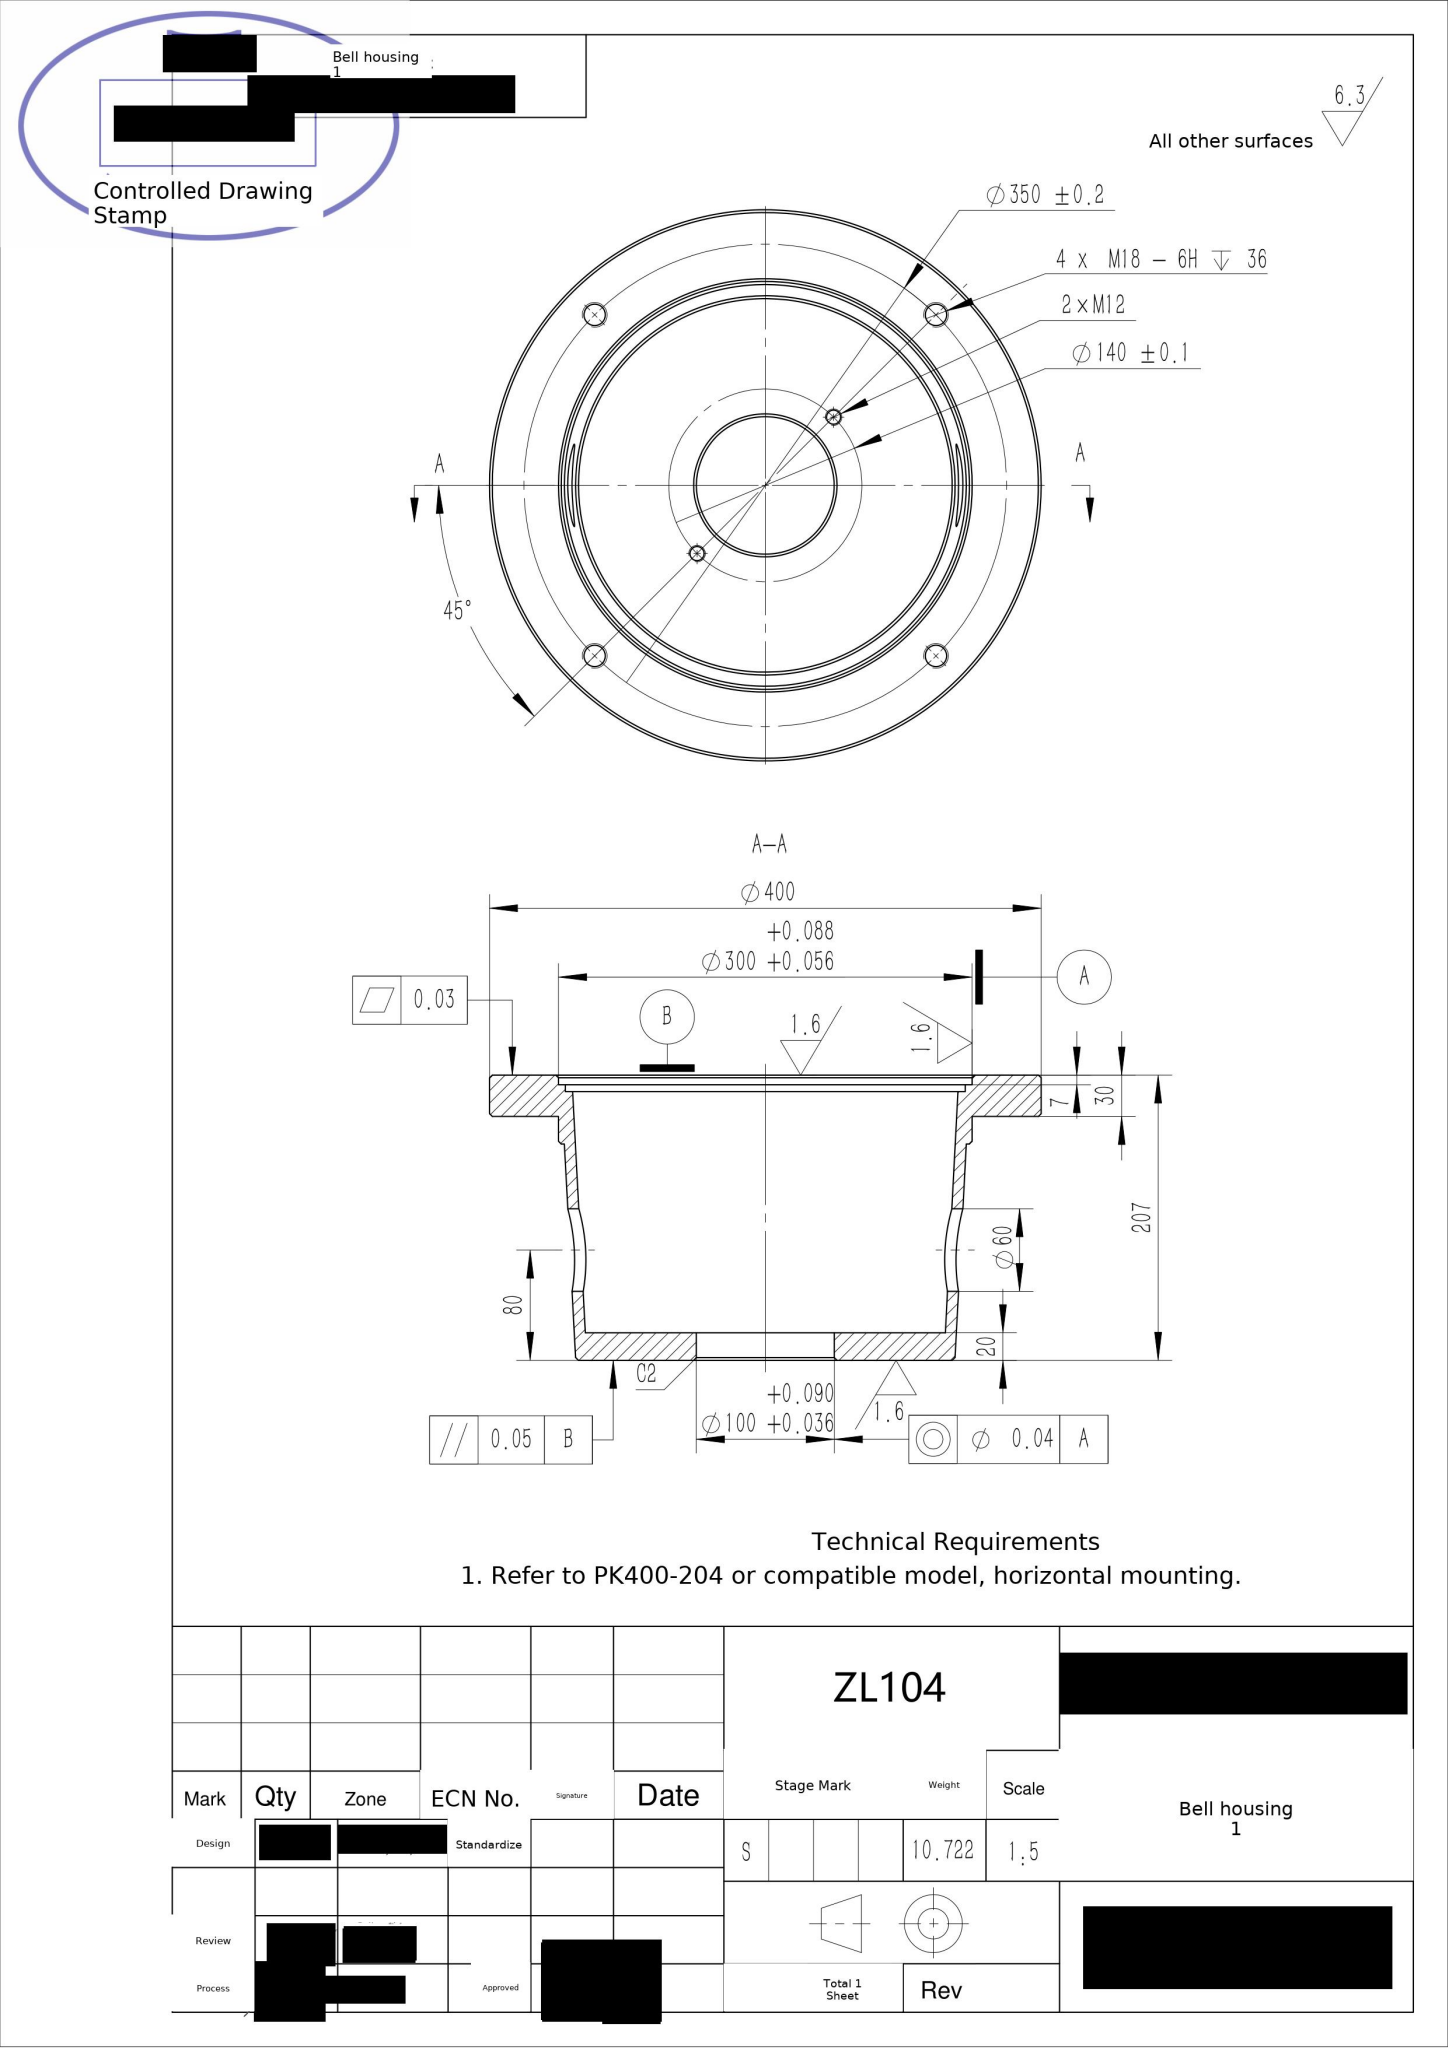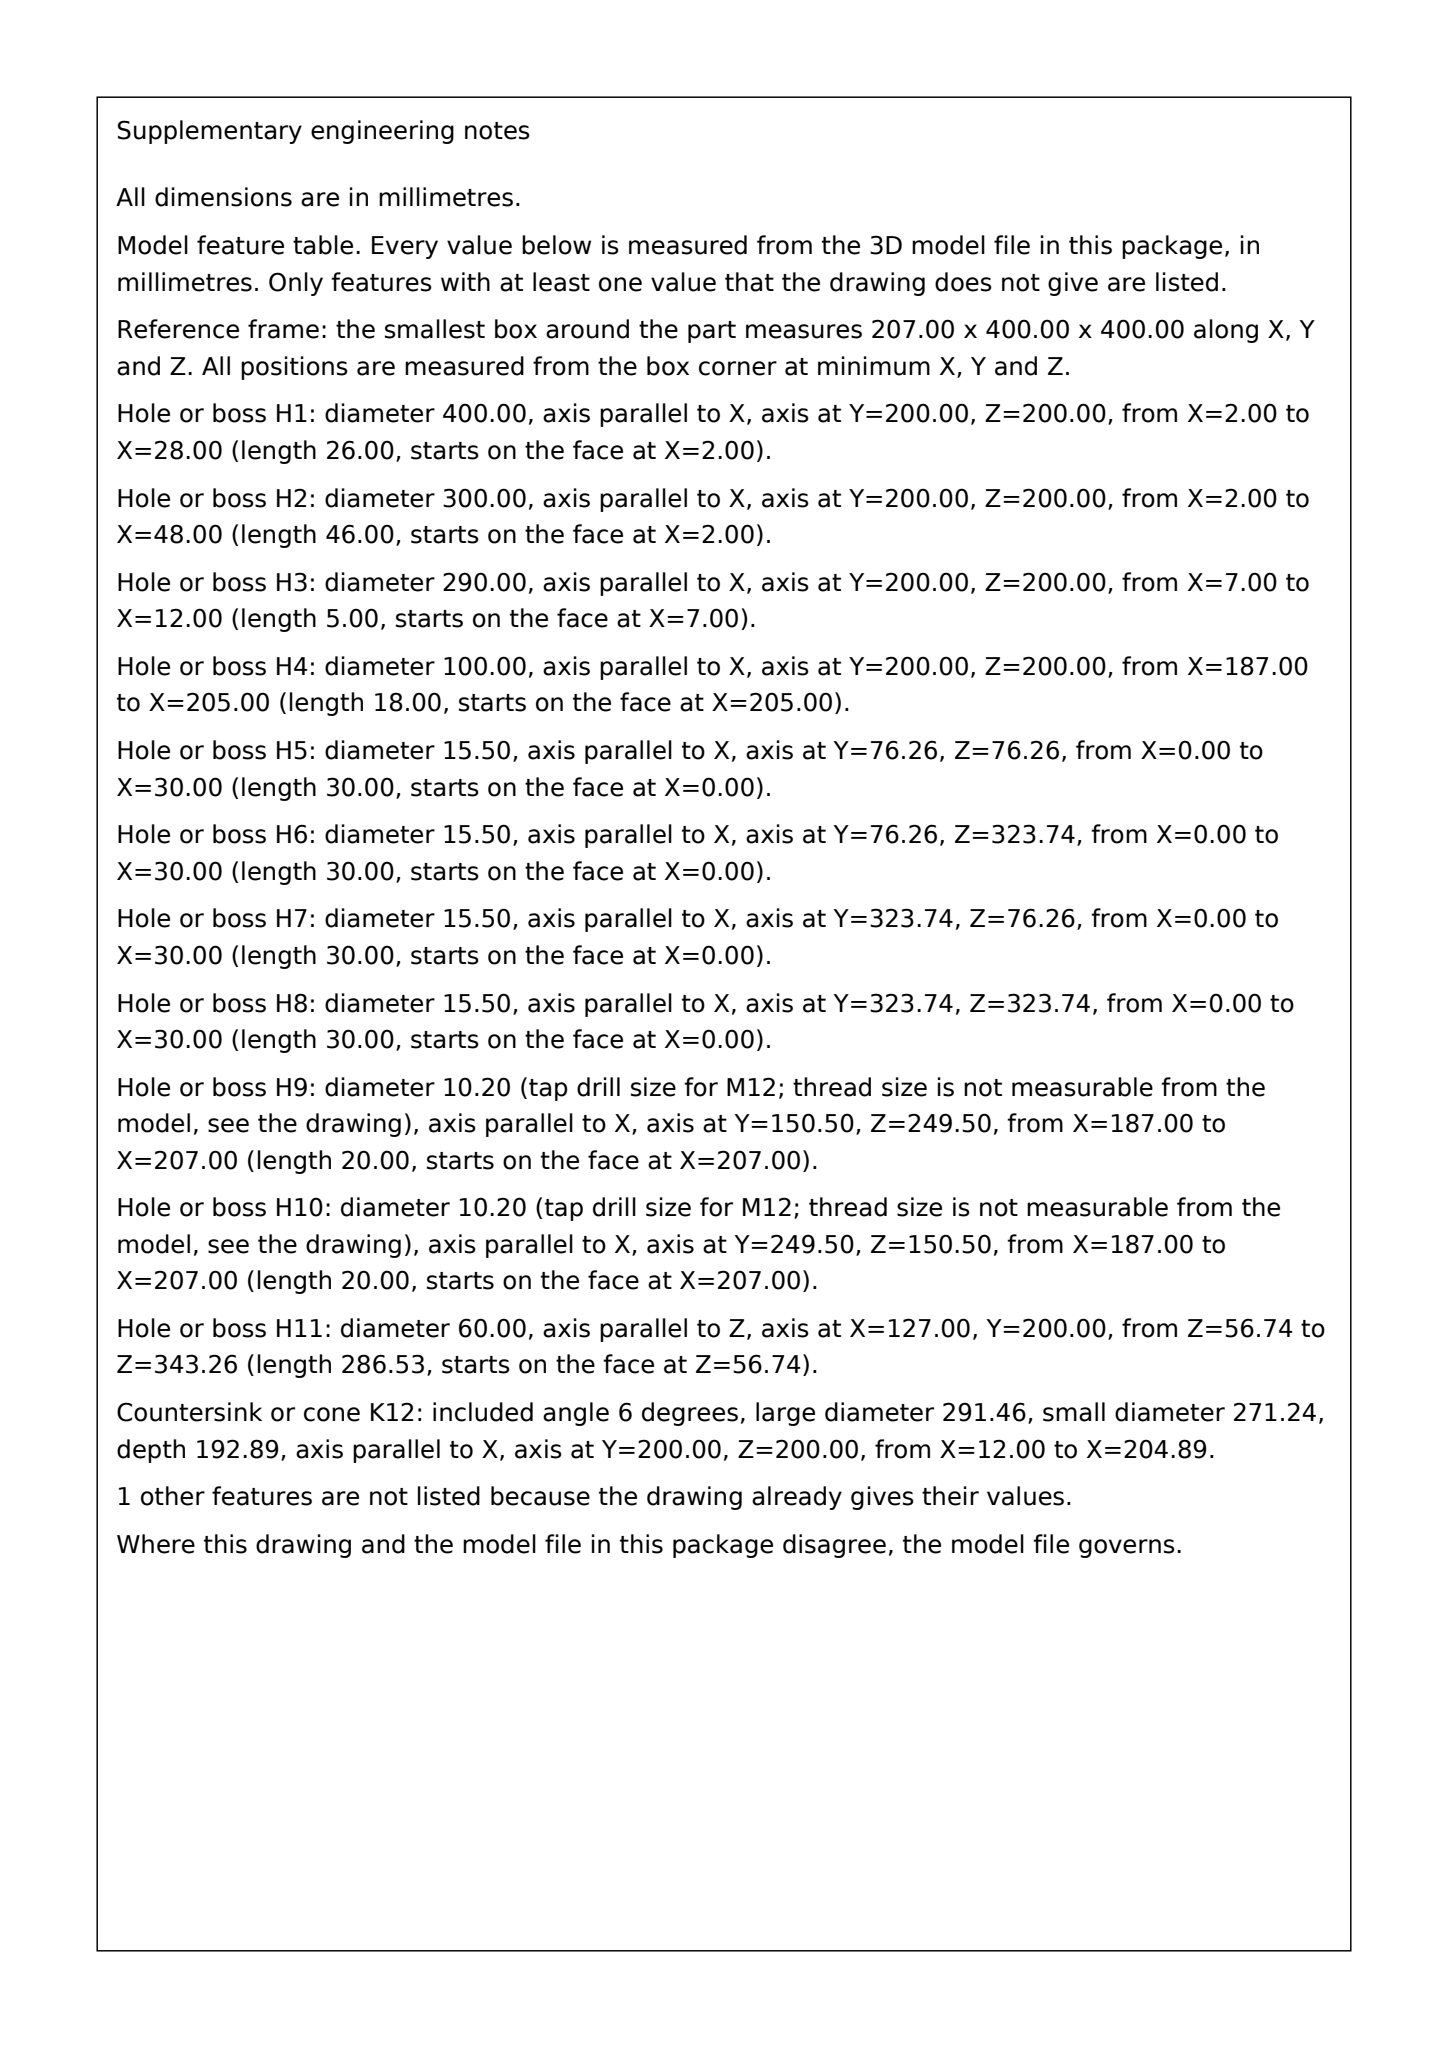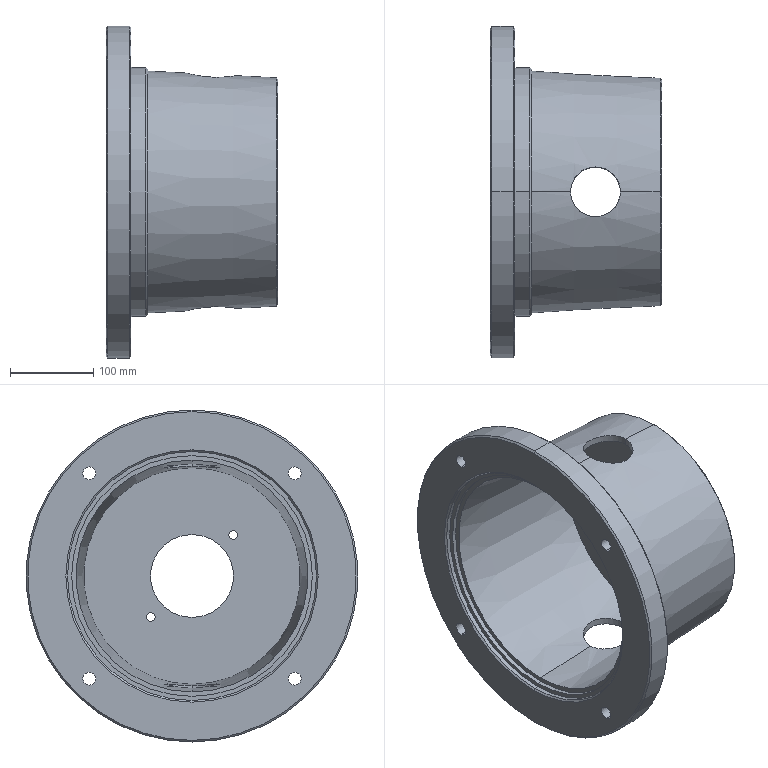Part | SolidWorks | mm | material ZL104 | 1 solid | 49 faces | box 207 x 400 x 400 mm | volume 3971271 mm3 | cylinder 26 | cone 16 | plane 7 | commonest cylinder face diameters 15.5 x8 10.2 x4 60 x4 300 x4 290 x2 100 x2 400 x2